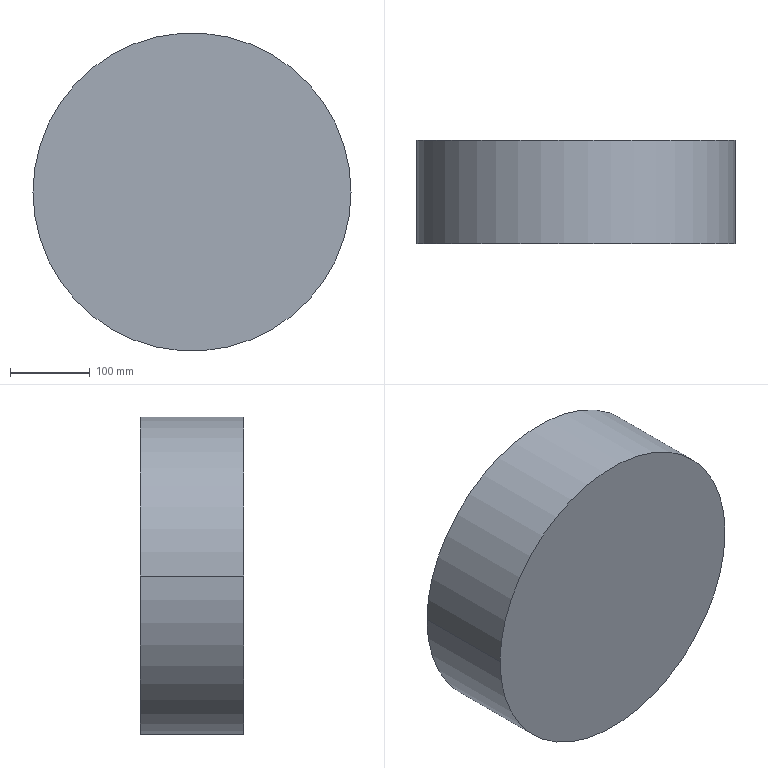Component | SolidWorks | 400ShockAbsorbingPad-1 | 1 solid | 8 faces | box 400 x 130 x 400 mm | volume 16266148 mm3 | cylinder 4 | cone 2 | plane 2 | commonest cylinder face diameters 400 x2 32 x2 | material Plain Carbon Steel
STEP:
#1=CARTESIAN_POINT('',(-36.811,-2.756,9.252));
#2=VERTEX_POINT('',#1);
#3=CARTESIAN_POINT('',(-21.063,-2.756,9.252));
#4=VERTEX_POINT('',#3);
#5=CARTESIAN_POINT('',(-28.937,-2.756,9.252));
#6=DIRECTION('',(0.,-1.,0.));
#7=DIRECTION('',(-1.,0.,0.));
#8=AXIS2_PLACEMENT_3D('',#5,#6,#7);
#9=CIRCLE('',#8,7.874);
#10=EDGE_CURVE('',#2,#4,#9,.T.);
#11=ORIENTED_EDGE('',*,*,#10,.T.);
#12=CARTESIAN_POINT('',(-21.063,-7.874,9.252));
#13=VERTEX_POINT('',#12);
#14=CARTESIAN_POINT('',(-21.063,-2.756,9.252));
#15=DIRECTION('',(0.,-1.,0.));
#16=VECTOR('',#15,39.37);
#17=LINE('',#14,#16);
#18=EDGE_CURVE('',#4,#13,#17,.T.);
#19=ORIENTED_EDGE('',*,*,#18,.T.);
#20=CARTESIAN_POINT('',(-36.811,-7.874,9.252));
#21=VERTEX_POINT('',#20);
#22=CARTESIAN_POINT('',(-28.937,-7.874,9.252));
#23=DIRECTION('',(0.,1.,0.));
#24=DIRECTION('',(-1.,0.,0.));
#25=AXIS2_PLACEMENT_3D('',#22,#23,#24);
#26=CIRCLE('',#25,7.874);
#27=EDGE_CURVE('',#13,#21,#26,.T.);
#28=ORIENTED_EDGE('',*,*,#27,.T.);
#29=CARTESIAN_POINT('',(-36.811,-2.756,9.252));
#30=DIRECTION('',(0.,-1.,0.));
#31=VECTOR('',#30,39.37);
#32=LINE('',#29,#31);
#33=EDGE_CURVE('',#2,#21,#32,.T.);
#34=ORIENTED_EDGE('',*,*,#33,.F.);
#35=EDGE_LOOP('',(#11,#19,#28,#34));
#36=FACE_OUTER_BOUND('',#35,.T.);
#37=CARTESIAN_POINT('',(-28.937,-2.756,9.252));
#38=DIRECTION('',(0.,-1.,0.));
#39=DIRECTION('',(-1.,0.,0.));
#40=AXIS2_PLACEMENT_3D('',#37,#38,#39);
#41=CYLINDRICAL_SURFACE('',#40,7.874);
#42=ADVANCED_FACE('',(#36),#41,.T.);
#43=CARTESIAN_POINT('',(-29.567,-6.063,9.252));
#44=VERTEX_POINT('',#43);
#45=CARTESIAN_POINT('',(-28.307,-6.063,9.252));
#46=VERTEX_POINT('',#45);
#47=CARTESIAN_POINT('',(-28.937,-6.063,9.252));
#48=DIRECTION('',(0.,1.,0.));
#49=DIRECTION('',(1.,0.,0.));
#50=AXIS2_PLACEMENT_3D('',#47,#48,#49);
#51=CIRCLE('',#50,0.6299);
#52=EDGE_CURVE('',#44,#46,#51,.T.);
#53=ORIENTED_EDGE('',*,*,#52,.F.);
#54=CARTESIAN_POINT('',(-29.567,-2.756,9.252));
#55=VERTEX_POINT('',#54);
#56=CARTESIAN_POINT('',(-29.567,-2.756,9.252));
#57=DIRECTION('',(0.,1.,0.));
#58=VECTOR('',#57,39.37);
#59=LINE('',#56,#58);
#60=EDGE_CURVE('',#44,#55,#59,.T.);
#61=ORIENTED_EDGE('',*,*,#60,.T.);
#62=CARTESIAN_POINT('',(-28.307,-2.756,9.252));
#63=VERTEX_POINT('',#62);
#64=CARTESIAN_POINT('',(-28.937,-2.756,9.252));
#65=DIRECTION('',(0.,-1.,0.));
#66=DIRECTION('',(1.,0.,0.));
#67=AXIS2_PLACEMENT_3D('',#64,#65,#66);
#68=CIRCLE('',#67,0.6299);
#69=EDGE_CURVE('',#63,#55,#68,.T.);
#70=ORIENTED_EDGE('',*,*,#69,.F.);
#71=CARTESIAN_POINT('',(-28.307,-2.756,9.252));
#72=DIRECTION('',(0.,1.,0.));
#73=VECTOR('',#72,39.37);
#74=LINE('',#71,#73);
#75=EDGE_CURVE('',#46,#63,#74,.T.);
#76=ORIENTED_EDGE('',*,*,#75,.F.);
#77=EDGE_LOOP('',(#53,#61,#70,#76));
#78=FACE_OUTER_BOUND('',#77,.T.);
#79=CARTESIAN_POINT('',(-28.937,-2.756,9.252));
#80=DIRECTION('',(0.,1.,0.));
#81=DIRECTION('',(1.,0.,0.));
#82=AXIS2_PLACEMENT_3D('',#79,#80,#81);
#83=CYLINDRICAL_SURFACE('',#82,0.6299);
#84=ADVANCED_FACE('',(#78),#83,.F.);
#85=CARTESIAN_POINT('',(-28.937,-6.441,9.252));
#86=VERTEX_POINT('',#85);
#87=CARTESIAN_POINT('',(-28.307,-6.063,9.252));
#88=DIRECTION('',(0.8572,0.515,0.));
#89=VECTOR('',#88,39.37);
#90=LINE('',#87,#89);
#91=EDGE_CURVE('',#86,#46,#90,.T.);
#92=ORIENTED_EDGE('',*,*,#91,.F.);
#93=CARTESIAN_POINT('',(-29.567,-6.063,9.252));
#94=DIRECTION('',(-0.8572,0.515,-0.));
#95=VECTOR('',#94,39.37);
#96=LINE('',#93,#95);
#97=EDGE_CURVE('',#86,#44,#96,.T.);
#98=ORIENTED_EDGE('',*,*,#97,.T.);
#99=ORIENTED_EDGE('',*,*,#52,.T.);
#100=EDGE_LOOP('',(#92,#98,#99));
#101=FACE_OUTER_BOUND('',#100,.T.);
#102=CARTESIAN_POINT('',(-28.937,-6.063,9.252));
#103=DIRECTION('',(0.,1.,0.));
#104=DIRECTION('',(1.,0.,0.));
#105=AXIS2_PLACEMENT_3D('',#102,#103,#104);
#106=CONICAL_SURFACE('',#105,0.6299,1.03);
#107=ADVANCED_FACE('',(#101),#106,.F.);
#108=CARTESIAN_POINT('',(-28.937,-7.874,9.252));
#109=DIRECTION('',(0.,1.,0.));
#110=DIRECTION('',(-1.,0.,0.));
#111=AXIS2_PLACEMENT_3D('',#108,#109,#110);
#112=CIRCLE('',#111,7.874);
#113=EDGE_CURVE('',#21,#13,#112,.T.);
#114=ORIENTED_EDGE('',*,*,#113,.F.);
#115=ORIENTED_EDGE('',*,*,#27,.F.);
#116=EDGE_LOOP('',(#114,#115));
#117=FACE_OUTER_BOUND('',#116,.T.);
#118=CARTESIAN_POINT('',(-28.937,-7.874,9.252));
#119=DIRECTION('',(0.,1.,0.));
#120=DIRECTION('',(1.,0.,0.));
#121=AXIS2_PLACEMENT_3D('',#118,#119,#120);
#122=PLANE('',#121);
#123=ADVANCED_FACE('',(#117),#122,.F.);
#124=ORIENTED_EDGE('',*,*,#18,.F.);
#125=CARTESIAN_POINT('',(-28.937,-2.756,9.252));
#126=DIRECTION('',(0.,-1.,0.));
#127=DIRECTION('',(-1.,0.,0.));
#128=AXIS2_PLACEMENT_3D('',#125,#126,#127);
#129=CIRCLE('',#128,7.874);
#130=EDGE_CURVE('',#4,#2,#129,.T.);
#131=ORIENTED_EDGE('',*,*,#130,.T.);
#132=ORIENTED_EDGE('',*,*,#33,.T.);
#133=ORIENTED_EDGE('',*,*,#113,.T.);
#134=EDGE_LOOP('',(#124,#131,#132,#133));
#135=FACE_OUTER_BOUND('',#134,.T.);
#136=CARTESIAN_POINT('',(-28.937,-2.756,9.252));
#137=DIRECTION('',(0.,-1.,0.));
#138=DIRECTION('',(-1.,0.,0.));
#139=AXIS2_PLACEMENT_3D('',#136,#137,#138);
#140=CYLINDRICAL_SURFACE('',#139,7.874);
#141=ADVANCED_FACE('',(#135),#140,.T.);
#142=ORIENTED_EDGE('',*,*,#10,.F.);
#143=ORIENTED_EDGE('',*,*,#130,.F.);
#144=EDGE_LOOP('',(#142,#143));
#145=FACE_OUTER_BOUND('',#144,.T.);
#146=ORIENTED_EDGE('',*,*,#69,.T.);
#147=CARTESIAN_POINT('',(-28.937,-2.756,9.252));
#148=DIRECTION('',(0.,-1.,0.));
#149=DIRECTION('',(1.,0.,0.));
#150=AXIS2_PLACEMENT_3D('',#147,#148,#149);
#151=CIRCLE('',#150,0.6299);
#152=EDGE_CURVE('',#55,#63,#151,.T.);
#153=ORIENTED_EDGE('',*,*,#152,.T.);
#154=EDGE_LOOP('',(#146,#153));
#155=FACE_BOUND('',#154,.T.);
#156=CARTESIAN_POINT('',(-28.937,-2.756,9.252));
#157=DIRECTION('',(0.,1.,0.));
#158=DIRECTION('',(1.,0.,0.));
#159=AXIS2_PLACEMENT_3D('',#156,#157,#158);
#160=PLANE('',#159);
#161=ADVANCED_FACE('',(#145,#155),#160,.T.);
#162=ORIENTED_EDGE('',*,*,#60,.F.);
#163=CARTESIAN_POINT('',(-28.937,-6.063,9.252));
#164=DIRECTION('',(0.,1.,0.));
#165=DIRECTION('',(1.,0.,0.));
#166=AXIS2_PLACEMENT_3D('',#163,#164,#165);
#167=CIRCLE('',#166,0.6299);
#168=EDGE_CURVE('',#46,#44,#167,.T.);
#169=ORIENTED_EDGE('',*,*,#168,.F.);
#170=ORIENTED_EDGE('',*,*,#75,.T.);
#171=ORIENTED_EDGE('',*,*,#152,.F.);
#172=EDGE_LOOP('',(#162,#169,#170,#171));
#173=FACE_OUTER_BOUND('',#172,.T.);
#174=CARTESIAN_POINT('',(-28.937,-2.756,9.252));
#175=DIRECTION('',(0.,1.,0.));
#176=DIRECTION('',(1.,0.,0.));
#177=AXIS2_PLACEMENT_3D('',#174,#175,#176);
#178=CYLINDRICAL_SURFACE('',#177,0.6299);
#179=ADVANCED_FACE('',(#173),#178,.F.);
#180=ORIENTED_EDGE('',*,*,#97,.F.);
#181=ORIENTED_EDGE('',*,*,#91,.T.);
#182=ORIENTED_EDGE('',*,*,#168,.T.);
#183=EDGE_LOOP('',(#180,#181,#182));
#184=FACE_OUTER_BOUND('',#183,.T.);
#185=CARTESIAN_POINT('',(-28.937,-6.063,9.252));
#186=DIRECTION('',(0.,1.,0.));
#187=DIRECTION('',(1.,0.,0.));
#188=AXIS2_PLACEMENT_3D('',#185,#186,#187);
#189=CONICAL_SURFACE('',#188,0.6299,1.03);
#190=ADVANCED_FACE('',(#184),#189,.F.);
#191=CLOSED_SHELL('',(#42,#84,#107,#123,#141,#161,#179,#190));
#192=MANIFOLD_SOLID_BREP('',#191);
#193=CARTESIAN_POINT('',(0.,0.,0.));
#194=DIRECTION('',(0.,0.,1.));
#195=DIRECTION('',(1.,0.,0.));
#196=AXIS2_PLACEMENT_3D('',#193,#194,#195);
#197=(LENGTH_UNIT()NAMED_UNIT(*)SI_UNIT($,.METRE.));
#198=LENGTH_MEASURE_WITH_UNIT(LENGTH_MEASURE(0.0254),#197);
#199=DIMENSIONAL_EXPONENTS(1.,0.,0.,0.,0.,0.,0.);
#200=(CONVERSION_BASED_UNIT('',#198)LENGTH_UNIT()NAMED_UNIT(#199));
#201=UNCERTAINTY_MEASURE_WITH_UNIT(LENGTH_MEASURE(0.00001),#200,'','');
#202=(NAMED_UNIT(*)PLANE_ANGLE_UNIT()SI_UNIT($,.RADIAN.));
#203=(NAMED_UNIT(*)SI_UNIT($,.STERADIAN.)SOLID_ANGLE_UNIT());
#204=(GEOMETRIC_REPRESENTATION_CONTEXT(3)GLOBAL_UNCERTAINTY_ASSIGNED_CONTEXT((#201))GLOBAL_UNIT_ASSIGNED_CONTEXT((#200,#202,#203))REPRESENTATION_CONTEXT('',''));
#205=ADVANCED_BREP_SHAPE_REPRESENTATION('',(#192,#196),#204);
#206=COLOUR_RGB('',0.7922,0.8196,0.9333);
#207=FILL_AREA_STYLE_COLOUR('',#206);
#208=FILL_AREA_STYLE('',(#207));
#209=SURFACE_STYLE_FILL_AREA(#208);
#210=SURFACE_SIDE_STYLE('',(#209));
#211=SURFACE_STYLE_USAGE(.BOTH.,#210);
#212=PRESENTATION_STYLE_ASSIGNMENT((#211));
#213=STYLED_ITEM('',(#212),#192);
#214=PRESENTATION_LAYER_ASSIGNMENT('','',(#213));
#215=(LENGTH_UNIT()NAMED_UNIT(*)SI_UNIT($,.METRE.));
#216=LENGTH_MEASURE_WITH_UNIT(LENGTH_MEASURE(0.0254),#215);
#217=DIMENSIONAL_EXPONENTS(1.,0.,0.,0.,0.,0.,0.);
#218=(CONVERSION_BASED_UNIT('',#216)LENGTH_UNIT()NAMED_UNIT(#217));
#219=UNCERTAINTY_MEASURE_WITH_UNIT(LENGTH_MEASURE(0.00001),#218,'','');
#220=(NAMED_UNIT(*)PLANE_ANGLE_UNIT()SI_UNIT($,.RADIAN.));
#221=(NAMED_UNIT(*)SI_UNIT($,.STERADIAN.)SOLID_ANGLE_UNIT());
#222=(GEOMETRIC_REPRESENTATION_CONTEXT(3)GLOBAL_UNCERTAINTY_ASSIGNED_CONTEXT((#219))GLOBAL_UNIT_ASSIGNED_CONTEXT((#218,#220,#221))REPRESENTATION_CONTEXT('',''));
#223=MECHANICAL_DESIGN_GEOMETRIC_PRESENTATION_REPRESENTATION('',(#213),#222);